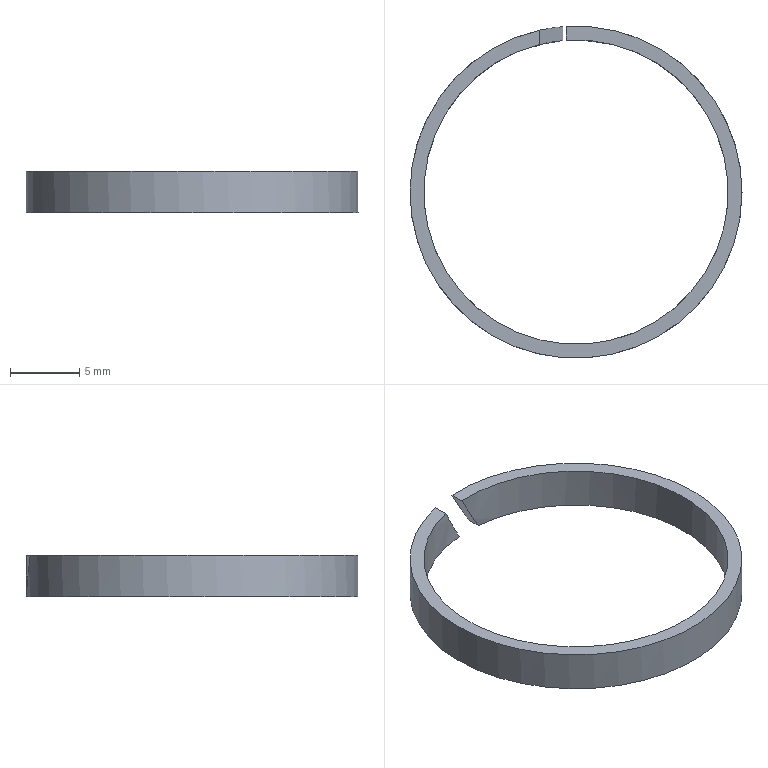Component | NX | PISTON_RING | 1 solid | 6 faces | box 24 x 24 x 3 mm | volume 211 mm3 | plane 4 | cylinder 2 | commonest cylinder face diameters 24 x1 22 x1
STEP:
#1=CARTESIAN_POINT('',(0.,0.,0.));
#2=DIRECTION('',(0.,0.,1.));
#3=DIRECTION('',(1.,0.,0.));
#4=AXIS2_PLACEMENT_3D('',#1,#2,#3);
#5=CARTESIAN_POINT('',(-0.9669,-25.039,23.));
#6=VERTEX_POINT('',#5);
#7=CARTESIAN_POINT('',(-2.63,-25.292,26.));
#8=VERTEX_POINT('',#7);
#9=CARTESIAN_POINT('',(-0.,-37.,21.256));
#10=DIRECTION('',(0.8746,0.,0.4848));
#11=DIRECTION('',(0.4848,0.,-0.8746));
#12=AXIS2_PLACEMENT_3D('',#9,#10,#11);
#13=ELLIPSE('',#12,24.752,12.);
#14=CARTESIAN_POINT('',(-0.,-37.,26.));
#15=DIRECTION('',(0.,0.,-1.));
#16=DIRECTION('',(0.,-1.,0.));
#17=AXIS2_PLACEMENT_3D('',#14,#15,#16);
#18=CYLINDRICAL_SURFACE('',#17,12.);
#19=CARTESIAN_POINT('',(9.344,3.));
#20=CARTESIAN_POINT('',(9.204,-0.));
#21=B_SPLINE_CURVE_WITH_KNOTS('',1,(#19,#20),.UNSPECIFIED.,.F.,.F.,(2,2),(1.651,1.792),.PIECEWISE_BEZIER_KNOTS.);
#22=(GEOMETRIC_REPRESENTATION_CONTEXT(2)PARAMETRIC_REPRESENTATION_CONTEXT()REPRESENTATION_CONTEXT('',''));
#23=DEFINITIONAL_REPRESENTATION('',(#21),#22);
#24=PCURVE('',#18,#23);
#25=CARTESIAN_POINT('',(-5.685,-17.,31.511));
#26=DIRECTION('',(-0.8746,0.,-0.4848));
#27=DIRECTION('',(-0.4848,0.,0.8746));
#28=AXIS2_PLACEMENT_3D('',#25,#26,#27);
#29=PLANE('',#28);
#30=CARTESIAN_POINT('',(-36.478,-20.));
#31=CARTESIAN_POINT('',(-36.478,0.7846));
#32=CARTESIAN_POINT('',(0.6504,-9.608));
#33=CARTESIAN_POINT('',(37.778,-20.));
#34=CARTESIAN_POINT('',(0.6504,-30.392));
#35=CARTESIAN_POINT('',(-36.478,-40.785));
#36=CARTESIAN_POINT('',(-36.478,-20.));
#37=(BOUNDED_CURVE()B_SPLINE_CURVE(2,(#30,#31,#32,#33,#34,#35,#36),.UNSPECIFIED.,.T.,.F.)B_SPLINE_CURVE_WITH_KNOTS((1,2,2,2,2,1),(-2.094,0.,2.094,4.189,6.283,8.378),.UNSPECIFIED.)CURVE()GEOMETRIC_REPRESENTATION_ITEM()RATIONAL_B_SPLINE_CURVE((1.,0.5,1.,0.5,1.,0.5,1.))REPRESENTATION_ITEM(''));
#38=(GEOMETRIC_REPRESENTATION_CONTEXT(2)PARAMETRIC_REPRESENTATION_CONTEXT()REPRESENTATION_CONTEXT('',''));
#39=DEFINITIONAL_REPRESENTATION('',(#37),#38);
#40=PCURVE('',#29,#39);
#41=SURFACE_CURVE('',#13,(#24,#40),.PCURVE_S1.);
#42=EDGE_CURVE('',#6,#8,#41,.T.);
#43=ORIENTED_EDGE('',*,*,#42,.F.);
#44=CARTESIAN_POINT('',(0.9669,-25.039,23.));
#45=VERTEX_POINT('',#44);
#46=CARTESIAN_POINT('',(-0.,-37.,23.));
#47=DIRECTION('',(0.,0.,-1.));
#48=DIRECTION('',(-0.,1.,0.));
#49=AXIS2_PLACEMENT_3D('',#46,#47,#48);
#50=CIRCLE('',#49,12.);
#51=CARTESIAN_POINT('',(3.142,3.));
#52=DIRECTION('',(1.,0.));
#53=VECTOR('',#52,1.);
#54=LINE('',#51,#53);
#55=(GEOMETRIC_REPRESENTATION_CONTEXT(2)PARAMETRIC_REPRESENTATION_CONTEXT()REPRESENTATION_CONTEXT('',''));
#56=DEFINITIONAL_REPRESENTATION('',(#54),#55);
#57=PCURVE('',#18,#56);
#58=CARTESIAN_POINT('',(-0.,-37.,23.));
#59=DIRECTION('',(0.,0.,-1.));
#60=DIRECTION('',(0.,-1.,0.));
#61=AXIS2_PLACEMENT_3D('',#58,#59,#60);
#62=PLANE('',#61);
#63=CARTESIAN_POINT('',(0.,0.));
#64=DIRECTION('',(-1.,0.));
#65=AXIS2_PLACEMENT_2D('',#63,#64);
#66=CIRCLE('',#65,12.);
#67=(GEOMETRIC_REPRESENTATION_CONTEXT(2)PARAMETRIC_REPRESENTATION_CONTEXT()REPRESENTATION_CONTEXT('',''));
#68=DEFINITIONAL_REPRESENTATION('',(#66),#67);
#69=PCURVE('',#62,#68);
#70=SURFACE_CURVE('',#50,(#57,#69),.PCURVE_S1.);
#71=EDGE_CURVE('',#45,#6,#70,.T.);
#72=ORIENTED_EDGE('',*,*,#71,.F.);
#73=CARTESIAN_POINT('',(-0.696,-25.02,26.));
#74=VERTEX_POINT('',#73);
#75=CARTESIAN_POINT('',(-0.,-37.,24.744));
#76=DIRECTION('',(-0.8746,0.,-0.4848));
#77=DIRECTION('',(0.4848,0.,-0.8746));
#78=AXIS2_PLACEMENT_3D('',#75,#76,#77);
#79=ELLIPSE('',#78,24.752,12.);
#80=CARTESIAN_POINT('',(3.084,-0.));
#81=CARTESIAN_POINT('',(3.222,3.));
#82=B_SPLINE_CURVE_WITH_KNOTS('',1,(#80,#81),.UNSPECIFIED.,.F.,.F.,(2,2),(4.654,4.793),.PIECEWISE_BEZIER_KNOTS.);
#83=(GEOMETRIC_REPRESENTATION_CONTEXT(2)PARAMETRIC_REPRESENTATION_CONTEXT()REPRESENTATION_CONTEXT('',''));
#84=DEFINITIONAL_REPRESENTATION('',(#82),#83);
#85=PCURVE('',#18,#84);
#86=CARTESIAN_POINT('',(5.685,-17.,14.489));
#87=DIRECTION('',(0.8746,0.,0.4848));
#88=DIRECTION('',(0.4848,0.,-0.8746));
#89=AXIS2_PLACEMENT_3D('',#86,#87,#88);
#90=PLANE('',#89);
#91=CARTESIAN_POINT('',(13.026,-20.));
#92=CARTESIAN_POINT('',(13.026,-40.785));
#93=CARTESIAN_POINT('',(-24.102,-30.392));
#94=CARTESIAN_POINT('',(-61.23,-20.));
#95=CARTESIAN_POINT('',(-24.102,-9.608));
#96=CARTESIAN_POINT('',(13.026,0.7846));
#97=CARTESIAN_POINT('',(13.026,-20.));
#98=(BOUNDED_CURVE()B_SPLINE_CURVE(2,(#91,#92,#93,#94,#95,#96,#97),.UNSPECIFIED.,.T.,.F.)B_SPLINE_CURVE_WITH_KNOTS((1,2,2,2,2,1),(-2.094,0.,2.094,4.189,6.283,8.378),.UNSPECIFIED.)CURVE()GEOMETRIC_REPRESENTATION_ITEM()RATIONAL_B_SPLINE_CURVE((1.,0.5,1.,0.5,1.,0.5,1.))REPRESENTATION_ITEM(''));
#99=(GEOMETRIC_REPRESENTATION_CONTEXT(2)PARAMETRIC_REPRESENTATION_CONTEXT()REPRESENTATION_CONTEXT('',''));
#100=DEFINITIONAL_REPRESENTATION('',(#98),#99);
#101=PCURVE('',#90,#100);
#102=SURFACE_CURVE('',#79,(#85,#101),.PCURVE_S1.);
#103=EDGE_CURVE('',#74,#45,#102,.T.);
#104=ORIENTED_EDGE('',*,*,#103,.F.);
#105=CARTESIAN_POINT('',(-0.,-37.,26.));
#106=DIRECTION('',(0.,0.,-1.));
#107=DIRECTION('',(-0.,1.,0.));
#108=AXIS2_PLACEMENT_3D('',#105,#106,#107);
#109=CIRCLE('',#108,12.);
#110=CARTESIAN_POINT('',(-3.142,0.));
#111=DIRECTION('',(1.,0.));
#112=VECTOR('',#111,1.);
#113=LINE('',#110,#112);
#114=(GEOMETRIC_REPRESENTATION_CONTEXT(2)PARAMETRIC_REPRESENTATION_CONTEXT()REPRESENTATION_CONTEXT('',''));
#115=DEFINITIONAL_REPRESENTATION('',(#113),#114);
#116=PCURVE('',#18,#115);
#117=CARTESIAN_POINT('',(-0.,-37.,26.));
#118=DIRECTION('',(0.,0.,-1.));
#119=DIRECTION('',(0.,-1.,0.));
#120=AXIS2_PLACEMENT_3D('',#117,#118,#119);
#121=PLANE('',#120);
#122=CARTESIAN_POINT('',(0.,0.));
#123=DIRECTION('',(-1.,0.));
#124=AXIS2_PLACEMENT_2D('',#122,#123);
#125=CIRCLE('',#124,12.);
#126=(GEOMETRIC_REPRESENTATION_CONTEXT(2)PARAMETRIC_REPRESENTATION_CONTEXT()REPRESENTATION_CONTEXT('',''));
#127=DEFINITIONAL_REPRESENTATION('',(#125),#126);
#128=PCURVE('',#121,#127);
#129=SURFACE_CURVE('',#109,(#116,#128),.PCURVE_S1.);
#130=EDGE_CURVE('',#74,#8,#129,.T.);
#131=ORIENTED_EDGE('',*,*,#130,.T.);
#132=EDGE_LOOP('',(#43,#72,#104,#131));
#133=FACE_BOUND('',#132,.T.);
#134=ADVANCED_FACE('',(#133),#18,.T.);
#135=CARTESIAN_POINT('',(-0.696,-26.022,26.));
#136=VERTEX_POINT('',#135);
#137=CARTESIAN_POINT('',(0.9669,-26.043,23.));
#138=VERTEX_POINT('',#137);
#139=CARTESIAN_POINT('',(-0.,-37.,24.744));
#140=DIRECTION('',(-0.8746,0.,-0.4848));
#141=DIRECTION('',(0.4848,0.,-0.8746));
#142=AXIS2_PLACEMENT_3D('',#139,#140,#141);
#143=ELLIPSE('',#142,22.689,11.);
#144=CARTESIAN_POINT('',(-0.,-37.,26.));
#145=DIRECTION('',(0.,0.,-1.));
#146=DIRECTION('',(0.,-1.,0.));
#147=AXIS2_PLACEMENT_3D('',#144,#145,#146);
#148=CYLINDRICAL_SURFACE('',#147,11.);
#149=CARTESIAN_POINT('',(3.078,-0.));
#150=CARTESIAN_POINT('',(3.23,3.));
#151=B_SPLINE_CURVE_WITH_KNOTS('',1,(#149,#150),.UNSPECIFIED.,.F.,.F.,(2,2),(4.649,4.8),.PIECEWISE_BEZIER_KNOTS.);
#152=(GEOMETRIC_REPRESENTATION_CONTEXT(2)PARAMETRIC_REPRESENTATION_CONTEXT()REPRESENTATION_CONTEXT('',''));
#153=DEFINITIONAL_REPRESENTATION('',(#151),#152);
#154=PCURVE('',#148,#153);
#155=CARTESIAN_POINT('',(10.964,-20.));
#156=CARTESIAN_POINT('',(10.964,-39.053));
#157=CARTESIAN_POINT('',(-23.07,-29.526));
#158=CARTESIAN_POINT('',(-57.104,-20.));
#159=CARTESIAN_POINT('',(-23.07,-10.474));
#160=CARTESIAN_POINT('',(10.964,-0.9474));
#161=CARTESIAN_POINT('',(10.964,-20.));
#162=(BOUNDED_CURVE()B_SPLINE_CURVE(2,(#155,#156,#157,#158,#159,#160,#161),.UNSPECIFIED.,.T.,.F.)B_SPLINE_CURVE_WITH_KNOTS((1,2,2,2,2,1),(-2.094,0.,2.094,4.189,6.283,8.378),.UNSPECIFIED.)CURVE()GEOMETRIC_REPRESENTATION_ITEM()RATIONAL_B_SPLINE_CURVE((1.,0.5,1.,0.5,1.,0.5,1.))REPRESENTATION_ITEM(''));
#163=(GEOMETRIC_REPRESENTATION_CONTEXT(2)PARAMETRIC_REPRESENTATION_CONTEXT()REPRESENTATION_CONTEXT('',''));
#164=DEFINITIONAL_REPRESENTATION('',(#162),#163);
#165=PCURVE('',#90,#164);
#166=SURFACE_CURVE('',#143,(#154,#165),.PCURVE_S1.);
#167=EDGE_CURVE('',#136,#138,#166,.T.);
#168=ORIENTED_EDGE('',*,*,#167,.F.);
#169=CARTESIAN_POINT('',(-2.63,-26.319,26.));
#170=VERTEX_POINT('',#169);
#171=CARTESIAN_POINT('',(-0.,-37.,26.));
#172=DIRECTION('',(0.,0.,-1.));
#173=DIRECTION('',(-0.,1.,0.));
#174=AXIS2_PLACEMENT_3D('',#171,#172,#173);
#175=CIRCLE('',#174,11.);
#176=CARTESIAN_POINT('',(-3.142,0.));
#177=DIRECTION('',(1.,0.));
#178=VECTOR('',#177,1.);
#179=LINE('',#176,#178);
#180=(GEOMETRIC_REPRESENTATION_CONTEXT(2)PARAMETRIC_REPRESENTATION_CONTEXT()REPRESENTATION_CONTEXT('',''));
#181=DEFINITIONAL_REPRESENTATION('',(#179),#180);
#182=PCURVE('',#148,#181);
#183=CARTESIAN_POINT('',(0.,0.));
#184=DIRECTION('',(-1.,0.));
#185=AXIS2_PLACEMENT_2D('',#183,#184);
#186=CIRCLE('',#185,11.);
#187=(GEOMETRIC_REPRESENTATION_CONTEXT(2)PARAMETRIC_REPRESENTATION_CONTEXT()REPRESENTATION_CONTEXT('',''));
#188=DEFINITIONAL_REPRESENTATION('',(#186),#187);
#189=PCURVE('',#121,#188);
#190=SURFACE_CURVE('',#175,(#182,#189),.PCURVE_S1.);
#191=EDGE_CURVE('',#136,#170,#190,.T.);
#192=ORIENTED_EDGE('',*,*,#191,.T.);
#193=CARTESIAN_POINT('',(-0.9669,-26.043,23.));
#194=VERTEX_POINT('',#193);
#195=CARTESIAN_POINT('',(-0.,-37.,21.256));
#196=DIRECTION('',(0.8746,0.,0.4848));
#197=DIRECTION('',(0.4848,0.,-0.8746));
#198=AXIS2_PLACEMENT_3D('',#195,#196,#197);
#199=ELLIPSE('',#198,22.689,11.);
#200=CARTESIAN_POINT('',(9.337,3.));
#201=CARTESIAN_POINT('',(9.183,-0.));
#202=B_SPLINE_CURVE_WITH_KNOTS('',1,(#200,#201),.UNSPECIFIED.,.F.,.F.,(2,2),(1.659,1.812),.PIECEWISE_BEZIER_KNOTS.);
#203=(GEOMETRIC_REPRESENTATION_CONTEXT(2)PARAMETRIC_REPRESENTATION_CONTEXT()REPRESENTATION_CONTEXT('',''));
#204=DEFINITIONAL_REPRESENTATION('',(#202),#203);
#205=PCURVE('',#148,#204);
#206=CARTESIAN_POINT('',(-34.415,-20.));
#207=CARTESIAN_POINT('',(-34.415,-0.9474));
#208=CARTESIAN_POINT('',(-0.3809,-10.474));
#209=CARTESIAN_POINT('',(33.653,-20.));
#210=CARTESIAN_POINT('',(-0.3809,-29.526));
#211=CARTESIAN_POINT('',(-34.415,-39.053));
#212=CARTESIAN_POINT('',(-34.415,-20.));
#213=(BOUNDED_CURVE()B_SPLINE_CURVE(2,(#206,#207,#208,#209,#210,#211,#212),.UNSPECIFIED.,.T.,.F.)B_SPLINE_CURVE_WITH_KNOTS((1,2,2,2,2,1),(-2.094,0.,2.094,4.189,6.283,8.378),.UNSPECIFIED.)CURVE()GEOMETRIC_REPRESENTATION_ITEM()RATIONAL_B_SPLINE_CURVE((1.,0.5,1.,0.5,1.,0.5,1.))REPRESENTATION_ITEM(''));
#214=(GEOMETRIC_REPRESENTATION_CONTEXT(2)PARAMETRIC_REPRESENTATION_CONTEXT()REPRESENTATION_CONTEXT('',''));
#215=DEFINITIONAL_REPRESENTATION('',(#213),#214);
#216=PCURVE('',#29,#215);
#217=SURFACE_CURVE('',#199,(#205,#216),.PCURVE_S1.);
#218=EDGE_CURVE('',#194,#170,#217,.T.);
#219=ORIENTED_EDGE('',*,*,#218,.F.);
#220=CARTESIAN_POINT('',(-0.,-37.,23.));
#221=DIRECTION('',(0.,0.,-1.));
#222=DIRECTION('',(-0.,1.,0.));
#223=AXIS2_PLACEMENT_3D('',#220,#221,#222);
#224=CIRCLE('',#223,11.);
#225=CARTESIAN_POINT('',(3.142,3.));
#226=DIRECTION('',(1.,0.));
#227=VECTOR('',#226,1.);
#228=LINE('',#225,#227);
#229=(GEOMETRIC_REPRESENTATION_CONTEXT(2)PARAMETRIC_REPRESENTATION_CONTEXT()REPRESENTATION_CONTEXT('',''));
#230=DEFINITIONAL_REPRESENTATION('',(#228),#229);
#231=PCURVE('',#148,#230);
#232=CARTESIAN_POINT('',(0.,0.));
#233=DIRECTION('',(-1.,0.));
#234=AXIS2_PLACEMENT_2D('',#232,#233);
#235=CIRCLE('',#234,11.);
#236=(GEOMETRIC_REPRESENTATION_CONTEXT(2)PARAMETRIC_REPRESENTATION_CONTEXT()REPRESENTATION_CONTEXT('',''));
#237=DEFINITIONAL_REPRESENTATION('',(#235),#236);
#238=PCURVE('',#62,#237);
#239=SURFACE_CURVE('',#224,(#231,#238),.PCURVE_S1.);
#240=EDGE_CURVE('',#138,#194,#239,.T.);
#241=ORIENTED_EDGE('',*,*,#240,.F.);
#242=EDGE_LOOP('',(#168,#192,#219,#241));
#243=FACE_BOUND('',#242,.F.);
#244=ADVANCED_FACE('',(#243),#148,.F.);
#245=ORIENTED_EDGE('',*,*,#191,.T.);
#246=CARTESIAN_POINT('',(-2.63,-37.,26.));
#247=DIRECTION('',(0.,1.,0.));
#248=VECTOR('',#247,1.);
#249=LINE('',#246,#248);
#250=CARTESIAN_POINT('',(0.,2.63));
#251=DIRECTION('',(-1.,0.));
#252=VECTOR('',#251,1.);
#253=LINE('',#250,#252);
#254=(GEOMETRIC_REPRESENTATION_CONTEXT(2)PARAMETRIC_REPRESENTATION_CONTEXT()REPRESENTATION_CONTEXT('',''));
#255=DEFINITIONAL_REPRESENTATION('',(#253),#254);
#256=PCURVE('',#121,#255);
#257=CARTESIAN_POINT('',(-6.301,-20.));
#258=DIRECTION('',(0.,1.));
#259=VECTOR('',#258,1.);
#260=LINE('',#257,#259);
#261=(GEOMETRIC_REPRESENTATION_CONTEXT(2)PARAMETRIC_REPRESENTATION_CONTEXT()REPRESENTATION_CONTEXT('',''));
#262=DEFINITIONAL_REPRESENTATION('',(#260),#261);
#263=PCURVE('',#29,#262);
#264=SURFACE_CURVE('',#249,(#256,#263),.PCURVE_S1.);
#265=EDGE_CURVE('',#170,#8,#264,.T.);
#266=ORIENTED_EDGE('',*,*,#265,.T.);
#267=ORIENTED_EDGE('',*,*,#130,.F.);
#268=CARTESIAN_POINT('',(-0.696,-37.,26.));
#269=DIRECTION('',(0.,-1.,0.));
#270=VECTOR('',#269,1.);
#271=LINE('',#268,#270);
#272=CARTESIAN_POINT('',(0.,0.696));
#273=DIRECTION('',(1.,0.));
#274=VECTOR('',#273,1.);
#275=LINE('',#272,#274);
#276=(GEOMETRIC_REPRESENTATION_CONTEXT(2)PARAMETRIC_REPRESENTATION_CONTEXT()REPRESENTATION_CONTEXT('',''));
#277=DEFINITIONAL_REPRESENTATION('',(#275),#276);
#278=PCURVE('',#121,#277);
#279=CARTESIAN_POINT('',(-13.161,-20.));
#280=DIRECTION('',(0.,-1.));
#281=VECTOR('',#280,1.);
#282=LINE('',#279,#281);
#283=(GEOMETRIC_REPRESENTATION_CONTEXT(2)PARAMETRIC_REPRESENTATION_CONTEXT()REPRESENTATION_CONTEXT('',''));
#284=DEFINITIONAL_REPRESENTATION('',(#282),#283);
#285=PCURVE('',#90,#284);
#286=SURFACE_CURVE('',#271,(#278,#285),.PCURVE_S1.);
#287=EDGE_CURVE('',#74,#136,#286,.T.);
#288=ORIENTED_EDGE('',*,*,#287,.T.);
#289=EDGE_LOOP('',(#245,#266,#267,#288));
#290=FACE_BOUND('',#289,.T.);
#291=ADVANCED_FACE('',(#290),#121,.F.);
#292=CARTESIAN_POINT('',(-0.9669,-37.,23.));
#293=DIRECTION('',(0.,1.,0.));
#294=VECTOR('',#293,1.);
#295=LINE('',#292,#294);
#296=CARTESIAN_POINT('',(0.,0.9669));
#297=DIRECTION('',(-1.,0.));
#298=VECTOR('',#297,1.);
#299=LINE('',#296,#298);
#300=(GEOMETRIC_REPRESENTATION_CONTEXT(2)PARAMETRIC_REPRESENTATION_CONTEXT()REPRESENTATION_CONTEXT('',''));
#301=DEFINITIONAL_REPRESENTATION('',(#299),#300);
#302=PCURVE('',#62,#301);
#303=CARTESIAN_POINT('',(-9.731,-20.));
#304=DIRECTION('',(0.,1.));
#305=VECTOR('',#304,1.);
#306=LINE('',#303,#305);
#307=(GEOMETRIC_REPRESENTATION_CONTEXT(2)PARAMETRIC_REPRESENTATION_CONTEXT()REPRESENTATION_CONTEXT('',''));
#308=DEFINITIONAL_REPRESENTATION('',(#306),#307);
#309=PCURVE('',#29,#308);
#310=SURFACE_CURVE('',#295,(#302,#309),.PCURVE_S1.);
#311=EDGE_CURVE('',#194,#6,#310,.T.);
#312=ORIENTED_EDGE('',*,*,#311,.F.);
#313=ORIENTED_EDGE('',*,*,#240,.F.);
#314=CARTESIAN_POINT('',(0.9669,-37.,23.));
#315=DIRECTION('',(0.,-1.,0.));
#316=VECTOR('',#315,1.);
#317=LINE('',#314,#316);
#318=CARTESIAN_POINT('',(0.,-0.9669));
#319=DIRECTION('',(1.,0.));
#320=VECTOR('',#319,1.);
#321=LINE('',#318,#320);
#322=(GEOMETRIC_REPRESENTATION_CONTEXT(2)PARAMETRIC_REPRESENTATION_CONTEXT()REPRESENTATION_CONTEXT('',''));
#323=DEFINITIONAL_REPRESENTATION('',(#321),#322);
#324=PCURVE('',#62,#323);
#325=CARTESIAN_POINT('',(-9.731,-20.));
#326=DIRECTION('',(0.,-1.));
#327=VECTOR('',#326,1.);
#328=LINE('',#325,#327);
#329=(GEOMETRIC_REPRESENTATION_CONTEXT(2)PARAMETRIC_REPRESENTATION_CONTEXT()REPRESENTATION_CONTEXT('',''));
#330=DEFINITIONAL_REPRESENTATION('',(#328),#329);
#331=PCURVE('',#90,#330);
#332=SURFACE_CURVE('',#317,(#324,#331),.PCURVE_S1.);
#333=EDGE_CURVE('',#45,#138,#332,.T.);
#334=ORIENTED_EDGE('',*,*,#333,.F.);
#335=ORIENTED_EDGE('',*,*,#71,.T.);
#336=EDGE_LOOP('',(#312,#313,#334,#335));
#337=FACE_BOUND('',#336,.T.);
#338=ADVANCED_FACE('',(#337),#62,.T.);
#339=ORIENTED_EDGE('',*,*,#103,.T.);
#340=ORIENTED_EDGE('',*,*,#333,.T.);
#341=ORIENTED_EDGE('',*,*,#167,.F.);
#342=ORIENTED_EDGE('',*,*,#287,.F.);
#343=EDGE_LOOP('',(#339,#340,#341,#342));
#344=FACE_BOUND('',#343,.T.);
#345=ADVANCED_FACE('',(#344),#90,.F.);
#346=ORIENTED_EDGE('',*,*,#218,.F.);
#347=ORIENTED_EDGE('',*,*,#311,.T.);
#348=ORIENTED_EDGE('',*,*,#42,.T.);
#349=ORIENTED_EDGE('',*,*,#265,.F.);
#350=EDGE_LOOP('',(#346,#347,#348,#349));
#351=FACE_BOUND('',#350,.T.);
#352=ADVANCED_FACE('',(#351),#29,.F.);
#353=CLOSED_SHELL('',(#134,#244,#291,#338,#345,#352));
#354=MANIFOLD_SOLID_BREP('',#353);
#355=(LENGTH_UNIT()NAMED_UNIT(*)SI_UNIT(.MILLI.,.METRE.));
#356=UNCERTAINTY_MEASURE_WITH_UNIT(LENGTH_MEASURE(0.005),#355,'','');
#357=(NAMED_UNIT(*)PLANE_ANGLE_UNIT()SI_UNIT($,.RADIAN.));
#358=(NAMED_UNIT(*)SI_UNIT($,.STERADIAN.)SOLID_ANGLE_UNIT());
#359=(GEOMETRIC_REPRESENTATION_CONTEXT(3)GLOBAL_UNCERTAINTY_ASSIGNED_CONTEXT((#356))GLOBAL_UNIT_ASSIGNED_CONTEXT((#355,#357,#358))REPRESENTATION_CONTEXT('',''));
#360=ADVANCED_BREP_SHAPE_REPRESENTATION('',(#4,#354),#359);